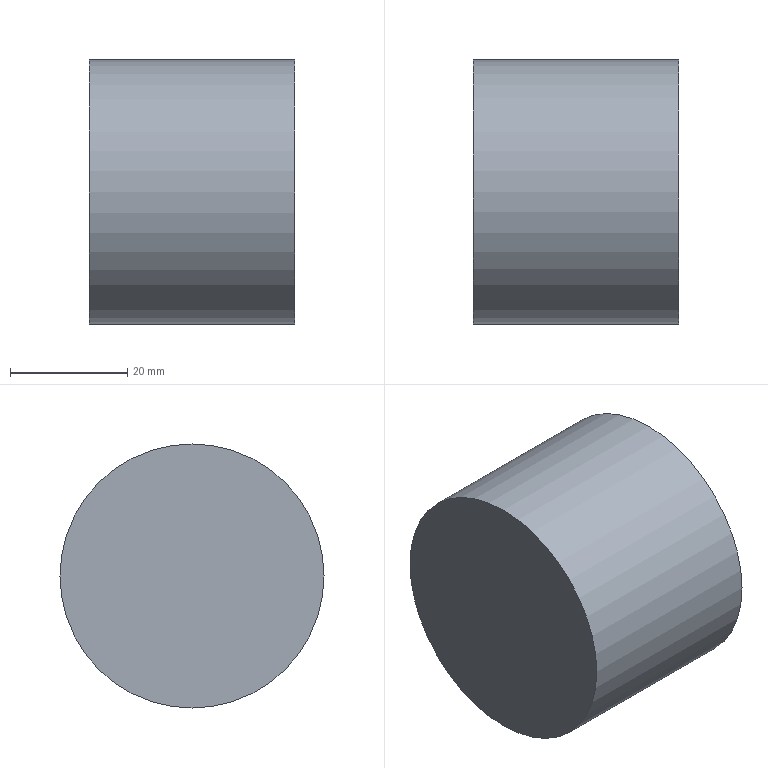Component | NX | HANDLE_SLEEVE | 1 solid | 5 faces | box 35 x 45 x 45 mm | volume 55420 mm3 | cylinder 2 | plane 2 | cone 1 | commonest cylinder face diameters 45 x1 5 x1
STEP:
#1=CARTESIAN_POINT('',(0.,0.,0.));
#2=DIRECTION('',(0.,0.,1.));
#3=DIRECTION('',(1.,0.,0.));
#4=AXIS2_PLACEMENT_3D('',#1,#2,#3);
#5=CARTESIAN_POINT('',(44.511,114.396,7.5));
#6=VERTEX_POINT('',#5);
#7=CARTESIAN_POINT('',(44.511,114.396,30.));
#8=DIRECTION('',(1.,0.,0.));
#9=DIRECTION('',(0.,0.,-1.));
#10=AXIS2_PLACEMENT_3D('',#7,#8,#9);
#11=CIRCLE('',#10,22.5);
#12=CARTESIAN_POINT('',(44.511,114.396,30.));
#13=DIRECTION('',(-1.,0.,0.));
#14=DIRECTION('',(0.,0.,1.));
#15=AXIS2_PLACEMENT_3D('',#12,#13,#14);
#16=CYLINDRICAL_SURFACE('',#15,22.5);
#17=CARTESIAN_POINT('',(9.425,0.));
#18=DIRECTION('',(-1.,0.));
#19=VECTOR('',#18,1.);
#20=LINE('',#17,#19);
#21=(GEOMETRIC_REPRESENTATION_CONTEXT(2)PARAMETRIC_REPRESENTATION_CONTEXT()REPRESENTATION_CONTEXT('',''));
#22=DEFINITIONAL_REPRESENTATION('',(#20),#21);
#23=PCURVE('',#16,#22);
#24=CARTESIAN_POINT('',(44.511,114.396,30.));
#25=DIRECTION('',(1.,0.,0.));
#26=DIRECTION('',(0.,0.,-1.));
#27=AXIS2_PLACEMENT_3D('',#24,#25,#26);
#28=PLANE('',#27);
#29=CARTESIAN_POINT('',(0.,0.));
#30=DIRECTION('',(1.,0.));
#31=AXIS2_PLACEMENT_2D('',#29,#30);
#32=CIRCLE('',#31,22.5);
#33=(GEOMETRIC_REPRESENTATION_CONTEXT(2)PARAMETRIC_REPRESENTATION_CONTEXT()REPRESENTATION_CONTEXT('',''));
#34=DEFINITIONAL_REPRESENTATION('',(#32),#33);
#35=PCURVE('',#28,#34);
#36=SURFACE_CURVE('',#11,(#23,#35),.PCURVE_S1.);
#37=EDGE_CURVE('',#6,#6,#36,.T.);
#38=ORIENTED_EDGE('',*,*,#37,.F.);
#39=CARTESIAN_POINT('',(9.511,114.396,7.5));
#40=VERTEX_POINT('',#39);
#41=CARTESIAN_POINT('',(44.511,114.396,7.5));
#42=CARTESIAN_POINT('',(9.511,114.396,7.5));
#43=B_SPLINE_CURVE_WITH_KNOTS('',1,(#41,#42),.UNSPECIFIED.,.F.,.F.,(2,2),(0.,35.),.PIECEWISE_BEZIER_KNOTS.);
#44=CARTESIAN_POINT('',(9.425,0.));
#45=DIRECTION('',(0.,1.));
#46=VECTOR('',#45,1.);
#47=LINE('',#44,#46);
#48=(GEOMETRIC_REPRESENTATION_CONTEXT(2)PARAMETRIC_REPRESENTATION_CONTEXT()REPRESENTATION_CONTEXT('',''));
#49=DEFINITIONAL_REPRESENTATION('',(#47),#48);
#50=PCURVE('',#16,#49);
#51=CARTESIAN_POINT('',(3.142,0.));
#52=DIRECTION('',(0.,1.));
#53=VECTOR('',#52,1.);
#54=LINE('',#51,#53);
#55=(GEOMETRIC_REPRESENTATION_CONTEXT(2)PARAMETRIC_REPRESENTATION_CONTEXT()REPRESENTATION_CONTEXT('',''));
#56=DEFINITIONAL_REPRESENTATION('',(#54),#55);
#57=PCURVE('',#16,#56);
#58=SEAM_CURVE('',#43,(#50,#57),.PCURVE_S1.);
#59=EDGE_CURVE('',#6,#40,#58,.T.);
#60=ORIENTED_EDGE('',*,*,#59,.T.);
#61=CARTESIAN_POINT('',(9.511,114.396,30.));
#62=DIRECTION('',(1.,0.,0.));
#63=DIRECTION('',(0.,0.,-1.));
#64=AXIS2_PLACEMENT_3D('',#61,#62,#63);
#65=CIRCLE('',#64,22.5);
#66=CARTESIAN_POINT('',(9.425,35.));
#67=DIRECTION('',(-1.,0.));
#68=VECTOR('',#67,1.);
#69=LINE('',#66,#68);
#70=(GEOMETRIC_REPRESENTATION_CONTEXT(2)PARAMETRIC_REPRESENTATION_CONTEXT()REPRESENTATION_CONTEXT('',''));
#71=DEFINITIONAL_REPRESENTATION('',(#69),#70);
#72=PCURVE('',#16,#71);
#73=CARTESIAN_POINT('',(9.511,114.396,30.));
#74=DIRECTION('',(1.,0.,0.));
#75=DIRECTION('',(0.,0.,-1.));
#76=AXIS2_PLACEMENT_3D('',#73,#74,#75);
#77=PLANE('',#76);
#78=CARTESIAN_POINT('',(0.,0.));
#79=DIRECTION('',(1.,0.));
#80=AXIS2_PLACEMENT_2D('',#78,#79);
#81=CIRCLE('',#80,22.5);
#82=(GEOMETRIC_REPRESENTATION_CONTEXT(2)PARAMETRIC_REPRESENTATION_CONTEXT()REPRESENTATION_CONTEXT('',''));
#83=DEFINITIONAL_REPRESENTATION('',(#81),#82);
#84=PCURVE('',#77,#83);
#85=SURFACE_CURVE('',#65,(#72,#84),.PCURVE_S1.);
#86=EDGE_CURVE('',#40,#40,#85,.T.);
#87=ORIENTED_EDGE('',*,*,#86,.T.);
#88=ORIENTED_EDGE('',*,*,#59,.F.);
#89=EDGE_LOOP('',(#38,#60,#87,#88));
#90=FACE_BOUND('',#89,.T.);
#91=ADVANCED_FACE('',(#90),#16,.T.);
#92=CARTESIAN_POINT('',(44.511,129.396,32.5));
#93=VERTEX_POINT('',#92);
#94=CARTESIAN_POINT('',(44.511,129.396,30.));
#95=DIRECTION('',(-1.,0.,0.));
#96=DIRECTION('',(0.,0.,1.));
#97=AXIS2_PLACEMENT_3D('',#94,#95,#96);
#98=CIRCLE('',#97,2.5);
#99=CARTESIAN_POINT('',(-2.5,15.));
#100=CARTESIAN_POINT('',(-2.5,19.33));
#101=CARTESIAN_POINT('',(1.25,17.165));
#102=CARTESIAN_POINT('',(5.,15.));
#103=CARTESIAN_POINT('',(1.25,12.835));
#104=CARTESIAN_POINT('',(-2.5,10.67));
#105=CARTESIAN_POINT('',(-2.5,15.));
#106=(BOUNDED_CURVE()B_SPLINE_CURVE(2,(#99,#100,#101,#102,#103,#104,#105),.UNSPECIFIED.,.T.,.F.)B_SPLINE_CURVE_WITH_KNOTS((1,2,2,2,2,1),(-2.094,0.,2.094,4.189,6.283,8.378),.UNSPECIFIED.)CURVE()GEOMETRIC_REPRESENTATION_ITEM()RATIONAL_B_SPLINE_CURVE((1.,0.5,1.,0.5,1.,0.5,1.))REPRESENTATION_ITEM(''));
#107=(GEOMETRIC_REPRESENTATION_CONTEXT(2)PARAMETRIC_REPRESENTATION_CONTEXT()REPRESENTATION_CONTEXT('',''));
#108=DEFINITIONAL_REPRESENTATION('',(#106),#107);
#109=PCURVE('',#28,#108);
#110=CARTESIAN_POINT('',(44.511,129.396,30.));
#111=DIRECTION('',(-1.,0.,0.));
#112=DIRECTION('',(0.,0.,1.));
#113=AXIS2_PLACEMENT_3D('',#110,#111,#112);
#114=CYLINDRICAL_SURFACE('',#113,2.5);
#115=CARTESIAN_POINT('',(0.,0.));
#116=DIRECTION('',(1.,0.));
#117=VECTOR('',#116,1.);
#118=LINE('',#115,#117);
#119=(GEOMETRIC_REPRESENTATION_CONTEXT(2)PARAMETRIC_REPRESENTATION_CONTEXT()REPRESENTATION_CONTEXT('',''));
#120=DEFINITIONAL_REPRESENTATION('',(#118),#119);
#121=PCURVE('',#114,#120);
#122=SURFACE_CURVE('',#98,(#109,#121),.PCURVE_S1.);
#123=EDGE_CURVE('',#93,#93,#122,.T.);
#124=ORIENTED_EDGE('',*,*,#123,.T.);
#125=EDGE_LOOP('',(#124));
#126=FACE_BOUND('',#125,.T.);
#127=ORIENTED_EDGE('',*,*,#37,.T.);
#128=EDGE_LOOP('',(#127));
#129=FACE_BOUND('',#128,.T.);
#130=ADVANCED_FACE('',(#126,#129),#28,.T.);
#131=ORIENTED_EDGE('',*,*,#86,.F.);
#132=EDGE_LOOP('',(#131));
#133=FACE_BOUND('',#132,.T.);
#134=ADVANCED_FACE('',(#133),#77,.F.);
#135=CARTESIAN_POINT('',(32.511,129.396,27.5));
#136=VERTEX_POINT('',#135);
#137=CARTESIAN_POINT('',(32.511,129.396,32.5));
#138=VERTEX_POINT('',#137);
#139=CARTESIAN_POINT('',(32.511,129.396,30.));
#140=DIRECTION('',(1.,0.,0.));
#141=DIRECTION('',(0.,0.,1.));
#142=AXIS2_PLACEMENT_3D('',#139,#140,#141);
#143=CIRCLE('',#142,2.5);
#144=CARTESIAN_POINT('',(32.511,129.396,30.));
#145=DIRECTION('',(1.,0.,0.));
#146=DIRECTION('',(0.,0.,-1.));
#147=AXIS2_PLACEMENT_3D('',#144,#145,#146);
#148=CONICAL_SURFACE('',#147,2.5,1.047);
#149=CARTESIAN_POINT('',(-3.142,0.));
#150=DIRECTION('',(1.,0.));
#151=VECTOR('',#150,1.);
#152=LINE('',#149,#151);
#153=(GEOMETRIC_REPRESENTATION_CONTEXT(2)PARAMETRIC_REPRESENTATION_CONTEXT()REPRESENTATION_CONTEXT('',''));
#154=DEFINITIONAL_REPRESENTATION('',(#152),#153);
#155=PCURVE('',#148,#154);
#156=CARTESIAN_POINT('',(6.283,12.));
#157=DIRECTION('',(-1.,0.));
#158=VECTOR('',#157,1.);
#159=LINE('',#156,#158);
#160=(GEOMETRIC_REPRESENTATION_CONTEXT(2)PARAMETRIC_REPRESENTATION_CONTEXT()REPRESENTATION_CONTEXT('',''));
#161=DEFINITIONAL_REPRESENTATION('',(#159),#160);
#162=PCURVE('',#114,#161);
#163=SURFACE_CURVE('',#143,(#155,#162),.PCURVE_S1.);
#164=EDGE_CURVE('',#136,#138,#163,.T.);
#165=ORIENTED_EDGE('',*,*,#164,.F.);
#166=CARTESIAN_POINT('',(31.067,129.396,30.));
#167=VERTEX_POINT('',#166);
#168=CARTESIAN_POINT('',(31.067,129.396,30.));
#169=CARTESIAN_POINT('',(32.511,129.396,27.5));
#170=B_SPLINE_CURVE_WITH_KNOTS('',1,(#168,#169),.UNSPECIFIED.,.F.,.F.,(2,2),(-2.887,0.),.PIECEWISE_BEZIER_KNOTS.);
#171=CARTESIAN_POINT('',(0.,0.));
#172=DIRECTION('',(0.,1.));
#173=VECTOR('',#172,1.);
#174=LINE('',#171,#173);
#175=(GEOMETRIC_REPRESENTATION_CONTEXT(2)PARAMETRIC_REPRESENTATION_CONTEXT()REPRESENTATION_CONTEXT('',''));
#176=DEFINITIONAL_REPRESENTATION('',(#174),#175);
#177=PCURVE('',#148,#176);
#178=CARTESIAN_POINT('',(6.283,0.));
#179=DIRECTION('',(0.,1.));
#180=VECTOR('',#179,1.);
#181=LINE('',#178,#180);
#182=(GEOMETRIC_REPRESENTATION_CONTEXT(2)PARAMETRIC_REPRESENTATION_CONTEXT()REPRESENTATION_CONTEXT('',''));
#183=DEFINITIONAL_REPRESENTATION('',(#181),#182);
#184=PCURVE('',#148,#183);
#185=SEAM_CURVE('',#170,(#177,#184),.PCURVE_S1.);
#186=EDGE_CURVE('',#167,#136,#185,.T.);
#187=ORIENTED_EDGE('',*,*,#186,.F.);
#188=ORIENTED_EDGE('',*,*,#186,.T.);
#189=CARTESIAN_POINT('',(32.511,129.396,30.));
#190=DIRECTION('',(1.,0.,0.));
#191=DIRECTION('',(0.,0.,1.));
#192=AXIS2_PLACEMENT_3D('',#189,#190,#191);
#193=CIRCLE('',#192,2.5);
#194=CARTESIAN_POINT('',(3.142,0.));
#195=DIRECTION('',(1.,0.));
#196=VECTOR('',#195,1.);
#197=LINE('',#194,#196);
#198=(GEOMETRIC_REPRESENTATION_CONTEXT(2)PARAMETRIC_REPRESENTATION_CONTEXT()REPRESENTATION_CONTEXT('',''));
#199=DEFINITIONAL_REPRESENTATION('',(#197),#198);
#200=PCURVE('',#148,#199);
#201=CARTESIAN_POINT('',(6.283,12.));
#202=DIRECTION('',(-1.,0.));
#203=VECTOR('',#202,1.);
#204=LINE('',#201,#203);
#205=(GEOMETRIC_REPRESENTATION_CONTEXT(2)PARAMETRIC_REPRESENTATION_CONTEXT()REPRESENTATION_CONTEXT('',''));
#206=DEFINITIONAL_REPRESENTATION('',(#204),#205);
#207=PCURVE('',#114,#206);
#208=SURFACE_CURVE('',#193,(#200,#207),.PCURVE_S1.);
#209=EDGE_CURVE('',#138,#136,#208,.T.);
#210=ORIENTED_EDGE('',*,*,#209,.F.);
#211=EDGE_LOOP('',(#165,#187,#188,#210));
#212=FACE_BOUND('',#211,.F.);
#213=ADVANCED_FACE('',(#212),#148,.F.);
#214=ORIENTED_EDGE('',*,*,#164,.T.);
#215=CARTESIAN_POINT('',(44.511,129.396,32.5));
#216=CARTESIAN_POINT('',(32.511,129.396,32.5));
#217=B_SPLINE_CURVE_WITH_KNOTS('',1,(#215,#216),.UNSPECIFIED.,.F.,.F.,(2,2),(0.,12.),.PIECEWISE_BEZIER_KNOTS.);
#218=CARTESIAN_POINT('',(0.,0.));
#219=DIRECTION('',(0.,1.));
#220=VECTOR('',#219,1.);
#221=LINE('',#218,#220);
#222=(GEOMETRIC_REPRESENTATION_CONTEXT(2)PARAMETRIC_REPRESENTATION_CONTEXT()REPRESENTATION_CONTEXT('',''));
#223=DEFINITIONAL_REPRESENTATION('',(#221),#222);
#224=PCURVE('',#114,#223);
#225=CARTESIAN_POINT('',(6.283,0.));
#226=DIRECTION('',(0.,1.));
#227=VECTOR('',#226,1.);
#228=LINE('',#225,#227);
#229=(GEOMETRIC_REPRESENTATION_CONTEXT(2)PARAMETRIC_REPRESENTATION_CONTEXT()REPRESENTATION_CONTEXT('',''));
#230=DEFINITIONAL_REPRESENTATION('',(#228),#229);
#231=PCURVE('',#114,#230);
#232=SEAM_CURVE('',#217,(#224,#231),.PCURVE_S1.);
#233=EDGE_CURVE('',#93,#138,#232,.T.);
#234=ORIENTED_EDGE('',*,*,#233,.F.);
#235=ORIENTED_EDGE('',*,*,#123,.T.);
#236=ORIENTED_EDGE('',*,*,#233,.T.);
#237=ORIENTED_EDGE('',*,*,#209,.T.);
#238=EDGE_LOOP('',(#214,#234,#235,#236,#237));
#239=FACE_BOUND('',#238,.F.);
#240=ADVANCED_FACE('',(#239),#114,.F.);
#241=CLOSED_SHELL('',(#91,#130,#134,#213,#240));
#242=MANIFOLD_SOLID_BREP('',#241);
#243=(LENGTH_UNIT()NAMED_UNIT(*)SI_UNIT(.MILLI.,.METRE.));
#244=UNCERTAINTY_MEASURE_WITH_UNIT(LENGTH_MEASURE(0.00001),#243,'','');
#245=(NAMED_UNIT(*)PLANE_ANGLE_UNIT()SI_UNIT($,.RADIAN.));
#246=(NAMED_UNIT(*)SI_UNIT($,.STERADIAN.)SOLID_ANGLE_UNIT());
#247=(GEOMETRIC_REPRESENTATION_CONTEXT(3)GLOBAL_UNCERTAINTY_ASSIGNED_CONTEXT((#244))GLOBAL_UNIT_ASSIGNED_CONTEXT((#243,#245,#246))REPRESENTATION_CONTEXT('',''));
#248=ADVANCED_BREP_SHAPE_REPRESENTATION('',(#4,#242),#247);